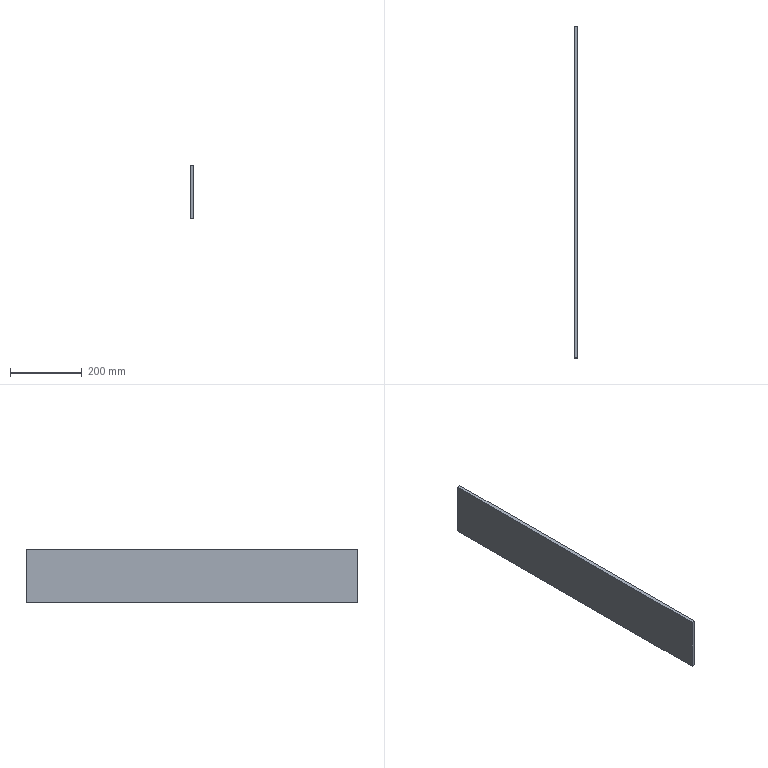Component | SolidWorks | SolderBoxFixingBracket-1 | 1 solid | 6 faces | box 10 x 925 x 150 mm | volume 1387500 mm3 | plane 6 | material Plain Carbon Steel
build123d program:
from build123d import *

# Parameters (mm, degrees)
SKETCH1_W           = 925
SKETCH1_H           = 150
BOSS_EXTRUDE1_DEPTH = 10


with BuildPart() as part:
    # Sketch1 → Boss-Extrude1 (new body)
    with BuildSketch(Plane.XY):
        Rectangle(SKETCH1_W, SKETCH1_H)
    extrude(amount=BOSS_EXTRUDE1_DEPTH)


solid = part.part

# Placed as in the assembly
solid = solid.moved(Location((-796.135, 72.093, 1088.102), (90, -90, 0)))
STEP:
#1=COLOUR_RGB('',0.7922,0.8196,0.9333);
#2=FILL_AREA_STYLE_COLOUR('',#1);
#3=FILL_AREA_STYLE('',(#2));
#4=SURFACE_STYLE_FILL_AREA(#3);
#5=SURFACE_SIDE_STYLE('',(#4));
#6=SURFACE_STYLE_USAGE(.BOTH.,#5);
#7=PRESENTATION_STYLE_ASSIGNMENT((#6));
#8=CARTESIAN_POINT('',(-31.738,-15.37,45.791));
#9=VERTEX_POINT('',#8);
#10=CARTESIAN_POINT('',(-31.738,-15.37,39.886));
#11=VERTEX_POINT('',#10);
#12=CARTESIAN_POINT('',(-31.738,-15.37,39.886));
#13=DIRECTION('',(-0.,0.,-1.));
#14=VECTOR('',#13,39.37);
#15=LINE('',#12,#14);
#16=EDGE_CURVE('',#9,#11,#15,.T.);
#17=ORIENTED_EDGE('',*,*,#16,.T.);
#18=CARTESIAN_POINT('',(-31.344,-15.37,39.886));
#19=VERTEX_POINT('',#18);
#20=CARTESIAN_POINT('',(-31.344,-15.37,39.886));
#21=DIRECTION('',(-1.,-0.,0.));
#22=VECTOR('',#21,39.37);
#23=LINE('',#20,#22);
#24=EDGE_CURVE('',#19,#11,#23,.T.);
#25=ORIENTED_EDGE('',*,*,#24,.F.);
#26=CARTESIAN_POINT('',(-31.344,-15.37,45.791));
#27=VERTEX_POINT('',#26);
#28=CARTESIAN_POINT('',(-31.344,-15.37,39.886));
#29=DIRECTION('',(-0.,0.,-1.));
#30=VECTOR('',#29,39.37);
#31=LINE('',#28,#30);
#32=EDGE_CURVE('',#27,#19,#31,.T.);
#33=ORIENTED_EDGE('',*,*,#32,.F.);
#34=CARTESIAN_POINT('',(-31.344,-15.37,45.791));
#35=DIRECTION('',(-1.,-0.,0.));
#36=VECTOR('',#35,39.37);
#37=LINE('',#34,#36);
#38=EDGE_CURVE('',#27,#9,#37,.T.);
#39=ORIENTED_EDGE('',*,*,#38,.T.);
#40=EDGE_LOOP('',(#17,#25,#33,#39));
#41=FACE_OUTER_BOUND('',#40,.T.);
#42=CARTESIAN_POINT('',(-31.344,-15.37,39.886));
#43=DIRECTION('',(-0.,1.,0.));
#44=DIRECTION('',(-1.,-0.,0.));
#45=AXIS2_PLACEMENT_3D('',#42,#43,#44);
#46=PLANE('',#45);
#47=ADVANCED_FACE('',(#41),#46,.F.);
#48=CARTESIAN_POINT('',(-31.738,21.047,39.886));
#49=VERTEX_POINT('',#48);
#50=CARTESIAN_POINT('',(-31.738,21.047,39.886));
#51=DIRECTION('',(-0.,1.,0.));
#52=VECTOR('',#51,39.37);
#53=LINE('',#50,#52);
#54=EDGE_CURVE('',#11,#49,#53,.T.);
#55=ORIENTED_EDGE('',*,*,#54,.T.);
#56=CARTESIAN_POINT('',(-31.344,21.047,39.886));
#57=VERTEX_POINT('',#56);
#58=CARTESIAN_POINT('',(-31.344,21.047,39.886));
#59=DIRECTION('',(-1.,-0.,0.));
#60=VECTOR('',#59,39.37);
#61=LINE('',#58,#60);
#62=EDGE_CURVE('',#57,#49,#61,.T.);
#63=ORIENTED_EDGE('',*,*,#62,.F.);
#64=CARTESIAN_POINT('',(-31.344,21.047,39.886));
#65=DIRECTION('',(-0.,1.,0.));
#66=VECTOR('',#65,39.37);
#67=LINE('',#64,#66);
#68=EDGE_CURVE('',#19,#57,#67,.T.);
#69=ORIENTED_EDGE('',*,*,#68,.F.);
#70=ORIENTED_EDGE('',*,*,#24,.T.);
#71=EDGE_LOOP('',(#55,#63,#69,#70));
#72=FACE_OUTER_BOUND('',#71,.T.);
#73=CARTESIAN_POINT('',(-31.344,21.047,39.886));
#74=DIRECTION('',(0.,-0.,1.));
#75=DIRECTION('',(0.,-1.,-0.));
#76=AXIS2_PLACEMENT_3D('',#73,#74,#75);
#77=PLANE('',#76);
#78=ADVANCED_FACE('',(#72),#77,.F.);
#79=CARTESIAN_POINT('',(-31.738,21.047,45.791));
#80=VERTEX_POINT('',#79);
#81=CARTESIAN_POINT('',(-31.738,21.047,39.886));
#82=DIRECTION('',(0.,-0.,1.));
#83=VECTOR('',#82,39.37);
#84=LINE('',#81,#83);
#85=EDGE_CURVE('',#49,#80,#84,.T.);
#86=ORIENTED_EDGE('',*,*,#85,.T.);
#87=CARTESIAN_POINT('',(-31.344,21.047,45.791));
#88=VERTEX_POINT('',#87);
#89=CARTESIAN_POINT('',(-31.344,21.047,45.791));
#90=DIRECTION('',(-1.,-0.,0.));
#91=VECTOR('',#90,39.37);
#92=LINE('',#89,#91);
#93=EDGE_CURVE('',#88,#80,#92,.T.);
#94=ORIENTED_EDGE('',*,*,#93,.F.);
#95=CARTESIAN_POINT('',(-31.344,21.047,39.886));
#96=DIRECTION('',(0.,-0.,1.));
#97=VECTOR('',#96,39.37);
#98=LINE('',#95,#97);
#99=EDGE_CURVE('',#57,#88,#98,.T.);
#100=ORIENTED_EDGE('',*,*,#99,.F.);
#101=ORIENTED_EDGE('',*,*,#62,.T.);
#102=EDGE_LOOP('',(#86,#94,#100,#101));
#103=FACE_OUTER_BOUND('',#102,.T.);
#104=CARTESIAN_POINT('',(-31.344,21.047,39.886));
#105=DIRECTION('',(0.,-1.,-0.));
#106=DIRECTION('',(1.,0.,-0.));
#107=AXIS2_PLACEMENT_3D('',#104,#105,#106);
#108=PLANE('',#107);
#109=ADVANCED_FACE('',(#103),#108,.F.);
#110=CARTESIAN_POINT('',(-31.738,21.047,45.791));
#111=DIRECTION('',(0.,-1.,-0.));
#112=VECTOR('',#111,39.37);
#113=LINE('',#110,#112);
#114=EDGE_CURVE('',#80,#9,#113,.T.);
#115=ORIENTED_EDGE('',*,*,#114,.T.);
#116=ORIENTED_EDGE('',*,*,#38,.F.);
#117=CARTESIAN_POINT('',(-31.344,21.047,45.791));
#118=DIRECTION('',(0.,-1.,-0.));
#119=VECTOR('',#118,39.37);
#120=LINE('',#117,#119);
#121=EDGE_CURVE('',#88,#27,#120,.T.);
#122=ORIENTED_EDGE('',*,*,#121,.F.);
#123=ORIENTED_EDGE('',*,*,#93,.T.);
#124=EDGE_LOOP('',(#115,#116,#122,#123));
#125=FACE_OUTER_BOUND('',#124,.T.);
#126=CARTESIAN_POINT('',(-31.344,21.047,45.791));
#127=DIRECTION('',(-0.,0.,-1.));
#128=DIRECTION('',(-0.,1.,0.));
#129=AXIS2_PLACEMENT_3D('',#126,#127,#128);
#130=PLANE('',#129);
#131=ADVANCED_FACE('',(#125),#130,.F.);
#132=ORIENTED_EDGE('',*,*,#32,.T.);
#133=ORIENTED_EDGE('',*,*,#68,.T.);
#134=ORIENTED_EDGE('',*,*,#99,.T.);
#135=ORIENTED_EDGE('',*,*,#121,.T.);
#136=EDGE_LOOP('',(#132,#133,#134,#135));
#137=FACE_OUTER_BOUND('',#136,.T.);
#138=CARTESIAN_POINT('',(-31.344,2.838,42.839));
#139=DIRECTION('',(1.,0.,-0.));
#140=DIRECTION('',(-0.,1.,0.));
#141=AXIS2_PLACEMENT_3D('',#138,#139,#140);
#142=PLANE('',#141);
#143=ADVANCED_FACE('',(#137),#142,.T.);
#144=ORIENTED_EDGE('',*,*,#16,.F.);
#145=ORIENTED_EDGE('',*,*,#114,.F.);
#146=ORIENTED_EDGE('',*,*,#85,.F.);
#147=ORIENTED_EDGE('',*,*,#54,.F.);
#148=EDGE_LOOP('',(#144,#145,#146,#147));
#149=FACE_OUTER_BOUND('',#148,.T.);
#150=CARTESIAN_POINT('',(-31.738,2.838,42.839));
#151=DIRECTION('',(1.,0.,-0.));
#152=DIRECTION('',(-0.,1.,0.));
#153=AXIS2_PLACEMENT_3D('',#150,#151,#152);
#154=PLANE('',#153);
#155=ADVANCED_FACE('',(#149),#154,.F.);
#156=CLOSED_SHELL('',(#47,#78,#109,#131,#143,#155));
#157=MANIFOLD_SOLID_BREP('',#156);
#158=STYLED_ITEM('',(#7),#157);
#159=PRESENTATION_LAYER_ASSIGNMENT('','',(#158));
#160=CARTESIAN_POINT('',(0.,0.,0.));
#161=DIRECTION('',(0.,0.,1.));
#162=DIRECTION('',(1.,0.,0.));
#163=AXIS2_PLACEMENT_3D('',#160,#161,#162);
#164=(LENGTH_UNIT()NAMED_UNIT(*)SI_UNIT($,.METRE.));
#165=LENGTH_MEASURE_WITH_UNIT(LENGTH_MEASURE(0.0254),#164);
#166=DIMENSIONAL_EXPONENTS(1.,0.,0.,0.,0.,0.,0.);
#167=(CONVERSION_BASED_UNIT('',#165)LENGTH_UNIT()NAMED_UNIT(#166));
#168=UNCERTAINTY_MEASURE_WITH_UNIT(LENGTH_MEASURE(0.00001),#167,'','');
#169=(NAMED_UNIT(*)PLANE_ANGLE_UNIT()SI_UNIT($,.RADIAN.));
#170=(NAMED_UNIT(*)SI_UNIT($,.STERADIAN.)SOLID_ANGLE_UNIT());
#171=(GEOMETRIC_REPRESENTATION_CONTEXT(3)GLOBAL_UNCERTAINTY_ASSIGNED_CONTEXT((#168))GLOBAL_UNIT_ASSIGNED_CONTEXT((#167,#169,#170))REPRESENTATION_CONTEXT('',''));
#172=ADVANCED_BREP_SHAPE_REPRESENTATION('',(#157,#163),#171);
#173=(LENGTH_UNIT()NAMED_UNIT(*)SI_UNIT($,.METRE.));
#174=LENGTH_MEASURE_WITH_UNIT(LENGTH_MEASURE(0.0254),#173);
#175=DIMENSIONAL_EXPONENTS(1.,0.,0.,0.,0.,0.,0.);
#176=(CONVERSION_BASED_UNIT('',#174)LENGTH_UNIT()NAMED_UNIT(#175));
#177=UNCERTAINTY_MEASURE_WITH_UNIT(LENGTH_MEASURE(0.00001),#176,'','');
#178=(NAMED_UNIT(*)PLANE_ANGLE_UNIT()SI_UNIT($,.RADIAN.));
#179=(NAMED_UNIT(*)SI_UNIT($,.STERADIAN.)SOLID_ANGLE_UNIT());
#180=(GEOMETRIC_REPRESENTATION_CONTEXT(3)GLOBAL_UNCERTAINTY_ASSIGNED_CONTEXT((#177))GLOBAL_UNIT_ASSIGNED_CONTEXT((#176,#178,#179))REPRESENTATION_CONTEXT('',''));
#181=MECHANICAL_DESIGN_GEOMETRIC_PRESENTATION_REPRESENTATION('',(#158),#180);